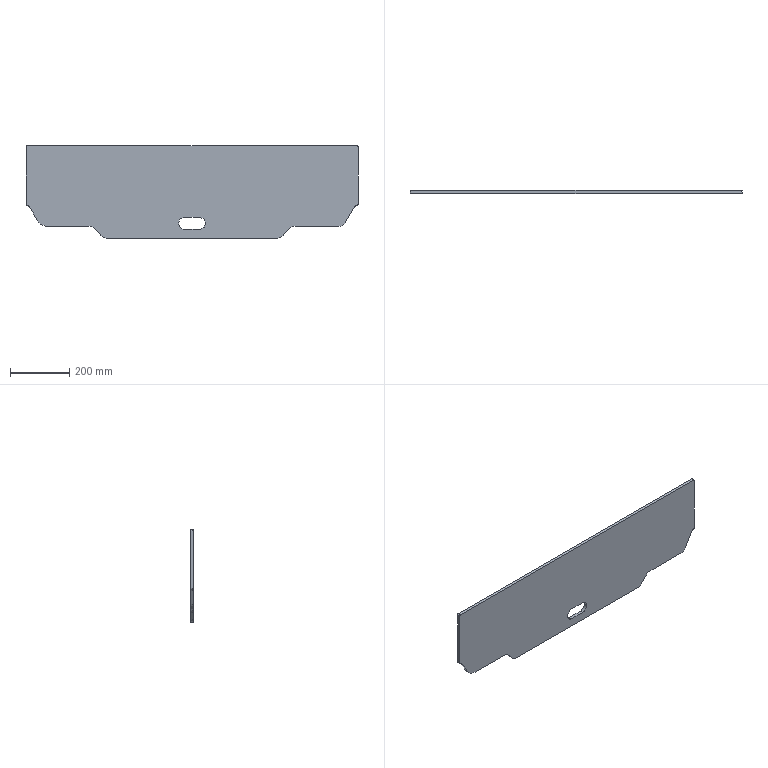Component | SolidWorks | FrontEndPlate,2-1 | 1 solid | 31 faces | box 1122 x 10 x 311.54 mm | volume 3226206 mm3 | plane 16 | cylinder 15 | commonest cylinder face diameters 50 x5 6 x4 40 x3 20 x2 80 x1 | material Q235
build123d program:
from build123d import *

# Parameters (mm, degrees)
BOSS_EXTRUDE1_DEPTH = 10


with BuildPart() as part:
    # Sketch1 → Boss-Extrude1 (new body)
    with BuildSketch(Plane.XY):
        with BuildLine():
            ThreePointArc((-290.657, -208.921), (-280.719, -210.981), (-272.419, -216.822))
            Line((-272.419, -216.822), (-249.734, -241.019))
            ThreePointArc((-249.734, -241.019), (-241.434, -246.861), (-231.495, -248.921))
            Line((-231.495, -248.921), (-59.652, -248.921))
            Line((-59.652, -248.921), (-13.084, -248.921))
            Line((-13.084, -248.921), (-2.185, -248.921))
            Line((-2.185, -248.921), (128.78, -248.921))
            Line((128.78, -248.921), (347.191, -248.921))
            ThreePointArc((347.191, -248.921), (357.129, -246.861), (365.43, -241.019))
            Line((365.43, -241.019), (388.114, -216.822))
            ThreePointArc((388.114, -216.822), (396.415, -210.981), (406.353, -208.921))
            Line((406.353, -208.921), (545.557, -208.921))
            ThreePointArc((545.557, -208.921), (565.355, -203.678), (579.962, -189.324))
            Line((579.962, -189.324), (607.86, -142.281))
            ThreePointArc((607.86, -142.281), (611.512, -138.692), (616.461, -137.382))
            Line((616.461, -137.382), (615.843, -137.382))
            ThreePointArc((615.843, -137.382), (617.964, -136.503), (618.843, -134.382))
            Line((618.843, -134.382), (618.843, 59.618))
            ThreePointArc((618.843, 59.618), (617.964, 61.74), (615.843, 62.618))
            Line((615.843, 62.618), (-240.657, 62.618))
            Line((-240.657, 62.618), (-500.157, 62.618))
            ThreePointArc((-500.157, 62.618), (-502.278, 61.74), (-503.157, 59.618))
            Line((-503.157, 59.618), (-503.157, -134.382))
            ThreePointArc((-503.157, -134.382), (-502.278, -136.503), (-500.157, -137.382))
            Line((-500.157, -137.382), (-500.765, -137.382))
            ThreePointArc((-500.765, -137.382), (-495.816, -138.692), (-492.164, -142.281))
            Line((-492.164, -142.281), (-460.397, -195.848))
            Line((-460.397, -195.848), (-459.43, -197.479))
            ThreePointArc((-459.43, -197.479), (-450.385, -205.875), (-438.426, -208.921))
            Line((-438.426, -208.921), (-290.657, -208.921))
        make_face()
        with BuildLine():
            ThreePointArc((32.848, -219.081), (12.85, -199.081), (32.848, -179.081))
            Line((32.848, -179.081), (82.848, -179.081))
            ThreePointArc((82.848, -179.081), (102.848, -199.081), (82.848, -219.081))
            Line((82.848, -219.081), (32.848, -219.081))
        make_face(mode=Mode.SUBTRACT)
    extrude(amount=BOSS_EXTRUDE1_DEPTH)


solid = part.part

# Placed as in the assembly
solid = solid.moved(Location((-759.311, 2402.474, 2748.087), (-90, 0, 180)))
STEP:
#1=COLOUR_RGB('',0.7922,0.8196,0.9333);
#2=FILL_AREA_STYLE_COLOUR('',#1);
#3=FILL_AREA_STYLE('',(#2));
#4=SURFACE_STYLE_FILL_AREA(#3);
#5=SURFACE_SIDE_STYLE('',(#4));
#6=SURFACE_STYLE_USAGE(.BOTH.,#5);
#7=PRESENTATION_STYLE_ASSIGNMENT((#6));
#8=CARTESIAN_POINT('',(-31.187,94.979,101.142));
#9=VERTEX_POINT('',#8);
#10=CARTESIAN_POINT('',(-30.4,94.979,100.355));
#11=VERTEX_POINT('',#10);
#12=CARTESIAN_POINT('',(-31.187,94.979,100.355));
#13=DIRECTION('',(-0.,1.,0.));
#14=DIRECTION('',(-1.,0.,0.));
#15=AXIS2_PLACEMENT_3D('',#12,#13,#14);
#16=CIRCLE('',#15,0.7874);
#17=EDGE_CURVE('',#9,#11,#16,.T.);
#18=ORIENTED_EDGE('',*,*,#17,.T.);
#19=CARTESIAN_POINT('',(-30.4,94.586,100.355));
#20=VERTEX_POINT('',#19);
#21=CARTESIAN_POINT('',(-30.4,94.979,100.355));
#22=DIRECTION('',(0.,-1.,-0.));
#23=VECTOR('',#22,39.37);
#24=LINE('',#21,#23);
#25=EDGE_CURVE('',#11,#20,#24,.T.);
#26=ORIENTED_EDGE('',*,*,#25,.T.);
#27=CARTESIAN_POINT('',(-31.187,94.586,101.142));
#28=VERTEX_POINT('',#27);
#29=CARTESIAN_POINT('',(-31.187,94.586,100.355));
#30=DIRECTION('',(-0.,1.,0.));
#31=DIRECTION('',(-1.,0.,0.));
#32=AXIS2_PLACEMENT_3D('',#29,#30,#31);
#33=CIRCLE('',#32,0.7874);
#34=EDGE_CURVE('',#28,#20,#33,.T.);
#35=ORIENTED_EDGE('',*,*,#34,.F.);
#36=CARTESIAN_POINT('',(-31.187,94.979,101.142));
#37=DIRECTION('',(0.,-1.,-0.));
#38=VECTOR('',#37,39.37);
#39=LINE('',#36,#38);
#40=EDGE_CURVE('',#9,#28,#39,.T.);
#41=ORIENTED_EDGE('',*,*,#40,.F.);
#42=EDGE_LOOP('',(#18,#26,#35,#41));
#43=FACE_OUTER_BOUND('',#42,.T.);
#44=CARTESIAN_POINT('',(-31.187,94.979,100.355));
#45=DIRECTION('',(0.,-1.,-0.));
#46=DIRECTION('',(1.,0.,-0.));
#47=AXIS2_PLACEMENT_3D('',#44,#45,#46);
#48=CYLINDRICAL_SURFACE('',#47,0.7874);
#49=ADVANCED_FACE('',(#43),#48,.F.);
#50=CARTESIAN_POINT('',(-54.258,94.586,110.54));
#51=VERTEX_POINT('',#50);
#52=CARTESIAN_POINT('',(-54.258,94.586,102.902));
#53=VERTEX_POINT('',#52);
#54=CARTESIAN_POINT('',(-54.258,94.586,108.192));
#55=DIRECTION('',(-0.,0.,-1.));
#56=VECTOR('',#55,39.37);
#57=LINE('',#54,#56);
#58=EDGE_CURVE('',#51,#53,#57,.T.);
#59=ORIENTED_EDGE('',*,*,#58,.F.);
#60=CARTESIAN_POINT('',(-54.258,94.979,110.54));
#61=VERTEX_POINT('',#60);
#62=CARTESIAN_POINT('',(-54.258,94.979,110.54));
#63=DIRECTION('',(0.,-1.,-0.));
#64=VECTOR('',#63,39.37);
#65=LINE('',#62,#64);
#66=EDGE_CURVE('',#61,#51,#65,.T.);
#67=ORIENTED_EDGE('',*,*,#66,.F.);
#68=CARTESIAN_POINT('',(-54.258,94.979,102.902));
#69=VERTEX_POINT('',#68);
#70=CARTESIAN_POINT('',(-54.258,94.979,108.192));
#71=DIRECTION('',(-0.,0.,-1.));
#72=VECTOR('',#71,39.37);
#73=LINE('',#70,#72);
#74=EDGE_CURVE('',#61,#69,#73,.T.);
#75=ORIENTED_EDGE('',*,*,#74,.T.);
#76=CARTESIAN_POINT('',(-54.258,94.979,102.902));
#77=DIRECTION('',(0.,-1.,-0.));
#78=VECTOR('',#77,39.37);
#79=LINE('',#76,#78);
#80=EDGE_CURVE('',#69,#53,#79,.T.);
#81=ORIENTED_EDGE('',*,*,#80,.T.);
#82=EDGE_LOOP('',(#59,#67,#75,#81));
#83=FACE_OUTER_BOUND('',#82,.T.);
#84=CARTESIAN_POINT('',(-54.258,94.979,108.192));
#85=DIRECTION('',(-1.,-0.,0.));
#86=DIRECTION('',(0.,-1.,-0.));
#87=AXIS2_PLACEMENT_3D('',#84,#85,#86);
#88=PLANE('',#87);
#89=ADVANCED_FACE('',(#83),#88,.T.);
#90=CARTESIAN_POINT('',(-54.14,94.586,110.658));
#91=VERTEX_POINT('',#90);
#92=CARTESIAN_POINT('',(-54.14,94.586,110.54));
#93=DIRECTION('',(-0.,1.,0.));
#94=DIRECTION('',(-1.,0.,0.));
#95=AXIS2_PLACEMENT_3D('',#92,#93,#94);
#96=CIRCLE('',#95,0.1181);
#97=EDGE_CURVE('',#51,#91,#96,.T.);
#98=ORIENTED_EDGE('',*,*,#97,.T.);
#99=CARTESIAN_POINT('',(-54.14,94.979,110.658));
#100=VERTEX_POINT('',#99);
#101=CARTESIAN_POINT('',(-54.14,94.979,110.658));
#102=DIRECTION('',(0.,-1.,-0.));
#103=VECTOR('',#102,39.37);
#104=LINE('',#101,#103);
#105=EDGE_CURVE('',#100,#91,#104,.T.);
#106=ORIENTED_EDGE('',*,*,#105,.F.);
#107=CARTESIAN_POINT('',(-54.14,94.979,110.54));
#108=DIRECTION('',(-0.,1.,0.));
#109=DIRECTION('',(-1.,0.,0.));
#110=AXIS2_PLACEMENT_3D('',#107,#108,#109);
#111=CIRCLE('',#110,0.1181);
#112=EDGE_CURVE('',#61,#100,#111,.T.);
#113=ORIENTED_EDGE('',*,*,#112,.F.);
#114=ORIENTED_EDGE('',*,*,#66,.T.);
#115=EDGE_LOOP('',(#98,#106,#113,#114));
#116=FACE_OUTER_BOUND('',#115,.T.);
#117=CARTESIAN_POINT('',(-54.14,94.979,110.54));
#118=DIRECTION('',(0.,-1.,-0.));
#119=DIRECTION('',(1.,0.,0.));
#120=AXIS2_PLACEMENT_3D('',#117,#118,#119);
#121=CYLINDRICAL_SURFACE('',#120,0.1181);
#122=ADVANCED_FACE('',(#116),#121,.T.);
#123=CARTESIAN_POINT('',(-10.203,94.586,110.658));
#124=VERTEX_POINT('',#123);
#125=CARTESIAN_POINT('',(-29.894,94.586,110.658));
#126=DIRECTION('',(1.,0.,-0.));
#127=VECTOR('',#126,39.37);
#128=LINE('',#125,#127);
#129=EDGE_CURVE('',#91,#124,#128,.T.);
#130=ORIENTED_EDGE('',*,*,#129,.T.);
#131=CARTESIAN_POINT('',(-10.203,94.979,110.658));
#132=VERTEX_POINT('',#131);
#133=CARTESIAN_POINT('',(-10.203,94.979,110.658));
#134=DIRECTION('',(0.,-1.,-0.));
#135=VECTOR('',#134,39.37);
#136=LINE('',#133,#135);
#137=EDGE_CURVE('',#132,#124,#136,.T.);
#138=ORIENTED_EDGE('',*,*,#137,.F.);
#139=CARTESIAN_POINT('',(-29.894,94.979,110.658));
#140=DIRECTION('',(1.,0.,-0.));
#141=VECTOR('',#140,39.37);
#142=LINE('',#139,#141);
#143=EDGE_CURVE('',#100,#132,#142,.T.);
#144=ORIENTED_EDGE('',*,*,#143,.F.);
#145=ORIENTED_EDGE('',*,*,#105,.T.);
#146=EDGE_LOOP('',(#130,#138,#144,#145));
#147=FACE_OUTER_BOUND('',#146,.T.);
#148=CARTESIAN_POINT('',(-29.894,94.979,110.658));
#149=DIRECTION('',(-0.,0.,-1.));
#150=DIRECTION('',(0.,-1.,-0.));
#151=AXIS2_PLACEMENT_3D('',#148,#149,#150);
#152=PLANE('',#151);
#153=ADVANCED_FACE('',(#147),#152,.F.);
#154=CARTESIAN_POINT('',(-10.085,94.586,110.54));
#155=VERTEX_POINT('',#154);
#156=CARTESIAN_POINT('',(-10.203,94.586,110.54));
#157=DIRECTION('',(-0.,1.,0.));
#158=DIRECTION('',(-1.,0.,0.));
#159=AXIS2_PLACEMENT_3D('',#156,#157,#158);
#160=CIRCLE('',#159,0.1181);
#161=EDGE_CURVE('',#124,#155,#160,.T.);
#162=ORIENTED_EDGE('',*,*,#161,.T.);
#163=CARTESIAN_POINT('',(-10.085,94.979,110.54));
#164=VERTEX_POINT('',#163);
#165=CARTESIAN_POINT('',(-10.085,94.979,110.54));
#166=DIRECTION('',(0.,-1.,-0.));
#167=VECTOR('',#166,39.37);
#168=LINE('',#165,#167);
#169=EDGE_CURVE('',#164,#155,#168,.T.);
#170=ORIENTED_EDGE('',*,*,#169,.F.);
#171=CARTESIAN_POINT('',(-10.203,94.979,110.54));
#172=DIRECTION('',(-0.,1.,0.));
#173=DIRECTION('',(-1.,0.,0.));
#174=AXIS2_PLACEMENT_3D('',#171,#172,#173);
#175=CIRCLE('',#174,0.1181);
#176=EDGE_CURVE('',#132,#164,#175,.T.);
#177=ORIENTED_EDGE('',*,*,#176,.F.);
#178=ORIENTED_EDGE('',*,*,#137,.T.);
#179=EDGE_LOOP('',(#162,#170,#177,#178));
#180=FACE_OUTER_BOUND('',#179,.T.);
#181=CARTESIAN_POINT('',(-10.203,94.979,110.54));
#182=DIRECTION('',(0.,-1.,-0.));
#183=DIRECTION('',(1.,0.,0.));
#184=AXIS2_PLACEMENT_3D('',#181,#182,#183);
#185=CYLINDRICAL_SURFACE('',#184,0.1181);
#186=ADVANCED_FACE('',(#180),#185,.T.);
#187=CARTESIAN_POINT('',(-10.085,94.586,102.902));
#188=VERTEX_POINT('',#187);
#189=CARTESIAN_POINT('',(-10.085,94.586,108.192));
#190=DIRECTION('',(0.,0.,-1.));
#191=VECTOR('',#190,39.37);
#192=LINE('',#189,#191);
#193=EDGE_CURVE('',#155,#188,#192,.T.);
#194=ORIENTED_EDGE('',*,*,#193,.T.);
#195=CARTESIAN_POINT('',(-10.085,94.979,102.902));
#196=VERTEX_POINT('',#195);
#197=CARTESIAN_POINT('',(-10.085,94.979,102.902));
#198=DIRECTION('',(0.,-1.,-0.));
#199=VECTOR('',#198,39.37);
#200=LINE('',#197,#199);
#201=EDGE_CURVE('',#196,#188,#200,.T.);
#202=ORIENTED_EDGE('',*,*,#201,.F.);
#203=CARTESIAN_POINT('',(-10.085,94.979,108.192));
#204=DIRECTION('',(0.,0.,-1.));
#205=VECTOR('',#204,39.37);
#206=LINE('',#203,#205);
#207=EDGE_CURVE('',#164,#196,#206,.T.);
#208=ORIENTED_EDGE('',*,*,#207,.F.);
#209=ORIENTED_EDGE('',*,*,#169,.T.);
#210=EDGE_LOOP('',(#194,#202,#208,#209));
#211=FACE_OUTER_BOUND('',#210,.T.);
#212=CARTESIAN_POINT('',(-10.085,94.979,108.192));
#213=DIRECTION('',(-1.,-0.,-0.));
#214=DIRECTION('',(-0.,-0.,1.));
#215=AXIS2_PLACEMENT_3D('',#212,#213,#214);
#216=PLANE('',#215);
#217=ADVANCED_FACE('',(#211),#216,.F.);
#218=CARTESIAN_POINT('',(-10.203,94.586,102.784));
#219=VERTEX_POINT('',#218);
#220=CARTESIAN_POINT('',(-10.203,94.586,102.902));
#221=DIRECTION('',(-0.,1.,0.));
#222=DIRECTION('',(-1.,0.,0.));
#223=AXIS2_PLACEMENT_3D('',#220,#221,#222);
#224=CIRCLE('',#223,0.1181);
#225=EDGE_CURVE('',#188,#219,#224,.T.);
#226=ORIENTED_EDGE('',*,*,#225,.T.);
#227=CARTESIAN_POINT('',(-10.203,94.979,102.784));
#228=VERTEX_POINT('',#227);
#229=CARTESIAN_POINT('',(-10.203,94.979,102.784));
#230=DIRECTION('',(0.,-1.,-0.));
#231=VECTOR('',#230,39.37);
#232=LINE('',#229,#231);
#233=EDGE_CURVE('',#228,#219,#232,.T.);
#234=ORIENTED_EDGE('',*,*,#233,.F.);
#235=CARTESIAN_POINT('',(-10.203,94.979,102.902));
#236=DIRECTION('',(-0.,1.,0.));
#237=DIRECTION('',(-1.,0.,0.));
#238=AXIS2_PLACEMENT_3D('',#235,#236,#237);
#239=CIRCLE('',#238,0.1181);
#240=EDGE_CURVE('',#196,#228,#239,.T.);
#241=ORIENTED_EDGE('',*,*,#240,.F.);
#242=ORIENTED_EDGE('',*,*,#201,.T.);
#243=EDGE_LOOP('',(#226,#234,#241,#242));
#244=FACE_OUTER_BOUND('',#243,.T.);
#245=CARTESIAN_POINT('',(-10.203,94.979,102.902));
#246=DIRECTION('',(0.,-1.,-0.));
#247=DIRECTION('',(1.,0.,0.));
#248=AXIS2_PLACEMENT_3D('',#245,#246,#247);
#249=CYLINDRICAL_SURFACE('',#248,0.1181);
#250=ADVANCED_FACE('',(#244),#249,.T.);
#251=CARTESIAN_POINT('',(-10.179,94.586,102.784));
#252=VERTEX_POINT('',#251);
#253=CARTESIAN_POINT('',(-29.894,94.586,102.784));
#254=DIRECTION('',(1.,0.,-0.));
#255=VECTOR('',#254,39.37);
#256=LINE('',#253,#255);
#257=EDGE_CURVE('',#219,#252,#256,.T.);
#258=ORIENTED_EDGE('',*,*,#257,.T.);
#259=CARTESIAN_POINT('',(-10.179,94.979,102.784));
#260=VERTEX_POINT('',#259);
#261=CARTESIAN_POINT('',(-10.179,94.979,102.784));
#262=DIRECTION('',(0.,-1.,-0.));
#263=VECTOR('',#262,39.37);
#264=LINE('',#261,#263);
#265=EDGE_CURVE('',#260,#252,#264,.T.);
#266=ORIENTED_EDGE('',*,*,#265,.F.);
#267=CARTESIAN_POINT('',(-29.894,94.979,102.784));
#268=DIRECTION('',(1.,0.,-0.));
#269=VECTOR('',#268,39.37);
#270=LINE('',#267,#269);
#271=EDGE_CURVE('',#228,#260,#270,.T.);
#272=ORIENTED_EDGE('',*,*,#271,.F.);
#273=ORIENTED_EDGE('',*,*,#233,.T.);
#274=EDGE_LOOP('',(#258,#266,#272,#273));
#275=FACE_OUTER_BOUND('',#274,.T.);
#276=CARTESIAN_POINT('',(-29.894,94.979,102.784));
#277=DIRECTION('',(-0.,0.,-1.));
#278=DIRECTION('',(0.,-1.,-0.));
#279=AXIS2_PLACEMENT_3D('',#276,#277,#278);
#280=PLANE('',#279);
#281=ADVANCED_FACE('',(#275),#280,.F.);
#282=CARTESIAN_POINT('',(-10.518,94.586,102.591));
#283=VERTEX_POINT('',#282);
#284=CARTESIAN_POINT('',(-10.179,94.586,102.39));
#285=DIRECTION('',(-0.,1.,0.));
#286=DIRECTION('',(-1.,0.,0.));
#287=AXIS2_PLACEMENT_3D('',#284,#285,#286);
#288=CIRCLE('',#287,0.3937);
#289=EDGE_CURVE('',#283,#252,#288,.T.);
#290=ORIENTED_EDGE('',*,*,#289,.F.);
#291=CARTESIAN_POINT('',(-10.518,94.979,102.591));
#292=VERTEX_POINT('',#291);
#293=CARTESIAN_POINT('',(-10.518,94.979,102.591));
#294=DIRECTION('',(0.,-1.,-0.));
#295=VECTOR('',#294,39.37);
#296=LINE('',#293,#295);
#297=EDGE_CURVE('',#292,#283,#296,.T.);
#298=ORIENTED_EDGE('',*,*,#297,.F.);
#299=CARTESIAN_POINT('',(-10.179,94.979,102.39));
#300=DIRECTION('',(-0.,1.,0.));
#301=DIRECTION('',(-1.,0.,0.));
#302=AXIS2_PLACEMENT_3D('',#299,#300,#301);
#303=CIRCLE('',#302,0.3937);
#304=EDGE_CURVE('',#292,#260,#303,.T.);
#305=ORIENTED_EDGE('',*,*,#304,.T.);
#306=ORIENTED_EDGE('',*,*,#265,.T.);
#307=EDGE_LOOP('',(#290,#298,#305,#306));
#308=FACE_OUTER_BOUND('',#307,.T.);
#309=CARTESIAN_POINT('',(-10.179,94.979,102.39));
#310=DIRECTION('',(0.,-1.,-0.));
#311=DIRECTION('',(1.,0.,0.));
#312=AXIS2_PLACEMENT_3D('',#309,#310,#311);
#313=CYLINDRICAL_SURFACE('',#312,0.3937);
#314=ADVANCED_FACE('',(#308),#313,.F.);
#315=CARTESIAN_POINT('',(-11.806,94.586,100.418));
#316=VERTEX_POINT('',#315);
#317=CARTESIAN_POINT('',(-13.101,94.586,98.234));
#318=DIRECTION('',(-0.5101,-0.,-0.8601));
#319=VECTOR('',#318,39.37);
#320=LINE('',#317,#319);
#321=EDGE_CURVE('',#283,#316,#320,.T.);
#322=ORIENTED_EDGE('',*,*,#321,.T.);
#323=CARTESIAN_POINT('',(-11.806,94.979,100.418));
#324=VERTEX_POINT('',#323);
#325=CARTESIAN_POINT('',(-11.806,94.979,100.418));
#326=DIRECTION('',(0.,-1.,-0.));
#327=VECTOR('',#326,39.37);
#328=LINE('',#325,#327);
#329=EDGE_CURVE('',#324,#316,#328,.T.);
#330=ORIENTED_EDGE('',*,*,#329,.F.);
#331=CARTESIAN_POINT('',(-13.101,94.979,98.234));
#332=DIRECTION('',(-0.5101,-0.,-0.8601));
#333=VECTOR('',#332,39.37);
#334=LINE('',#331,#333);
#335=EDGE_CURVE('',#292,#324,#334,.T.);
#336=ORIENTED_EDGE('',*,*,#335,.F.);
#337=ORIENTED_EDGE('',*,*,#297,.T.);
#338=EDGE_LOOP('',(#322,#330,#336,#337));
#339=FACE_OUTER_BOUND('',#338,.T.);
#340=CARTESIAN_POINT('',(-13.101,94.979,98.234));
#341=DIRECTION('',(-0.8601,-0.,0.5101));
#342=DIRECTION('',(0.5101,0.,0.8601));
#343=AXIS2_PLACEMENT_3D('',#340,#341,#342);
#344=PLANE('',#343);
#345=ADVANCED_FACE('',(#339),#344,.F.);
#346=CARTESIAN_POINT('',(-12.633,94.586,99.967));
#347=VERTEX_POINT('',#346);
#348=CARTESIAN_POINT('',(-12.633,94.586,100.951));
#349=DIRECTION('',(-0.,1.,0.));
#350=DIRECTION('',(-1.,-0.,0.));
#351=AXIS2_PLACEMENT_3D('',#348,#349,#350);
#352=CIRCLE('',#351,0.9843);
#353=EDGE_CURVE('',#316,#347,#352,.T.);
#354=ORIENTED_EDGE('',*,*,#353,.T.);
#355=CARTESIAN_POINT('',(-12.633,94.979,99.967));
#356=VERTEX_POINT('',#355);
#357=CARTESIAN_POINT('',(-12.633,94.979,99.967));
#358=DIRECTION('',(0.,-1.,-0.));
#359=VECTOR('',#358,39.37);
#360=LINE('',#357,#359);
#361=EDGE_CURVE('',#356,#347,#360,.T.);
#362=ORIENTED_EDGE('',*,*,#361,.F.);
#363=CARTESIAN_POINT('',(-12.633,94.979,100.951));
#364=DIRECTION('',(-0.,1.,0.));
#365=DIRECTION('',(-1.,-0.,0.));
#366=AXIS2_PLACEMENT_3D('',#363,#364,#365);
#367=CIRCLE('',#366,0.9843);
#368=EDGE_CURVE('',#324,#356,#367,.T.);
#369=ORIENTED_EDGE('',*,*,#368,.F.);
#370=ORIENTED_EDGE('',*,*,#329,.T.);
#371=EDGE_LOOP('',(#354,#362,#369,#370));
#372=FACE_OUTER_BOUND('',#371,.T.);
#373=CARTESIAN_POINT('',(-12.633,94.979,100.951));
#374=DIRECTION('',(0.,-1.,-0.));
#375=DIRECTION('',(1.,0.,-0.));
#376=AXIS2_PLACEMENT_3D('',#373,#374,#375);
#377=CYLINDRICAL_SURFACE('',#376,0.9843);
#378=ADVANCED_FACE('',(#372),#377,.T.);
#379=CARTESIAN_POINT('',(-18.451,94.586,99.967));
#380=VERTEX_POINT('',#379);
#381=CARTESIAN_POINT('',(-29.894,94.586,99.967));
#382=DIRECTION('',(-1.,-0.,0.));
#383=VECTOR('',#382,39.37);
#384=LINE('',#381,#383);
#385=EDGE_CURVE('',#347,#380,#384,.T.);
#386=ORIENTED_EDGE('',*,*,#385,.T.);
#387=CARTESIAN_POINT('',(-18.451,94.979,99.967));
#388=VERTEX_POINT('',#387);
#389=CARTESIAN_POINT('',(-18.451,94.979,99.967));
#390=DIRECTION('',(0.,-1.,-0.));
#391=VECTOR('',#390,39.37);
#392=LINE('',#389,#391);
#393=EDGE_CURVE('',#388,#380,#392,.T.);
#394=ORIENTED_EDGE('',*,*,#393,.F.);
#395=CARTESIAN_POINT('',(-29.894,94.979,99.967));
#396=DIRECTION('',(-1.,-0.,0.));
#397=VECTOR('',#396,39.37);
#398=LINE('',#395,#397);
#399=EDGE_CURVE('',#356,#388,#398,.T.);
#400=ORIENTED_EDGE('',*,*,#399,.F.);
#401=ORIENTED_EDGE('',*,*,#361,.T.);
#402=EDGE_LOOP('',(#386,#394,#400,#401));
#403=FACE_OUTER_BOUND('',#402,.T.);
#404=CARTESIAN_POINT('',(-29.894,94.979,99.967));
#405=DIRECTION('',(0.,-0.,1.));
#406=DIRECTION('',(1.,0.,-0.));
#407=AXIS2_PLACEMENT_3D('',#404,#405,#406);
#408=PLANE('',#407);
#409=ADVANCED_FACE('',(#403),#408,.F.);
#410=CARTESIAN_POINT('',(-19.169,94.586,99.656));
#411=VERTEX_POINT('',#410);
#412=CARTESIAN_POINT('',(-18.451,94.586,98.983));
#413=DIRECTION('',(-0.,1.,0.));
#414=DIRECTION('',(-1.,-0.,0.));
#415=AXIS2_PLACEMENT_3D('',#412,#413,#414);
#416=CIRCLE('',#415,0.9843);
#417=EDGE_CURVE('',#411,#380,#416,.T.);
#418=ORIENTED_EDGE('',*,*,#417,.F.);
#419=CARTESIAN_POINT('',(-19.169,94.979,99.656));
#420=VERTEX_POINT('',#419);
#421=CARTESIAN_POINT('',(-19.169,94.979,99.656));
#422=DIRECTION('',(0.,-1.,-0.));
#423=VECTOR('',#422,39.37);
#424=LINE('',#421,#423);
#425=EDGE_CURVE('',#420,#411,#424,.T.);
#426=ORIENTED_EDGE('',*,*,#425,.F.);
#427=CARTESIAN_POINT('',(-18.451,94.979,98.983));
#428=DIRECTION('',(-0.,1.,0.));
#429=DIRECTION('',(-1.,-0.,0.));
#430=AXIS2_PLACEMENT_3D('',#427,#428,#429);
#431=CIRCLE('',#430,0.9843);
#432=EDGE_CURVE('',#420,#388,#431,.T.);
#433=ORIENTED_EDGE('',*,*,#432,.T.);
#434=ORIENTED_EDGE('',*,*,#393,.T.);
#435=EDGE_LOOP('',(#418,#426,#433,#434));
#436=FACE_OUTER_BOUND('',#435,.T.);
#437=CARTESIAN_POINT('',(-18.451,94.979,98.983));
#438=DIRECTION('',(0.,-1.,-0.));
#439=DIRECTION('',(1.,0.,-0.));
#440=AXIS2_PLACEMENT_3D('',#437,#438,#439);
#441=CYLINDRICAL_SURFACE('',#440,0.9843);
#442=ADVANCED_FACE('',(#436),#441,.F.);
#443=CARTESIAN_POINT('',(-20.062,94.586,98.703));
#444=VERTEX_POINT('',#443);
#445=CARTESIAN_POINT('',(-19.927,94.586,98.848));
#446=DIRECTION('',(-0.6839,-0.,-0.7295));
#447=VECTOR('',#446,39.37);
#448=LINE('',#445,#447);
#449=EDGE_CURVE('',#411,#444,#448,.T.);
#450=ORIENTED_EDGE('',*,*,#449,.T.);
#451=CARTESIAN_POINT('',(-20.062,94.979,98.703));
#452=VERTEX_POINT('',#451);
#453=CARTESIAN_POINT('',(-20.062,94.979,98.703));
#454=DIRECTION('',(0.,-1.,-0.));
#455=VECTOR('',#454,39.37);
#456=LINE('',#453,#455);
#457=EDGE_CURVE('',#452,#444,#456,.T.);
#458=ORIENTED_EDGE('',*,*,#457,.F.);
#459=CARTESIAN_POINT('',(-19.927,94.979,98.848));
#460=DIRECTION('',(-0.6839,-0.,-0.7295));
#461=VECTOR('',#460,39.37);
#462=LINE('',#459,#461);
#463=EDGE_CURVE('',#420,#452,#462,.T.);
#464=ORIENTED_EDGE('',*,*,#463,.F.);
#465=ORIENTED_EDGE('',*,*,#425,.T.);
#466=EDGE_LOOP('',(#450,#458,#464,#465));
#467=FACE_OUTER_BOUND('',#466,.T.);
#468=CARTESIAN_POINT('',(-19.927,94.979,98.848));
#469=DIRECTION('',(-0.7295,-0.,0.6839));
#470=DIRECTION('',(0.6839,0.,0.7295));
#471=AXIS2_PLACEMENT_3D('',#468,#469,#470);
#472=PLANE('',#471);
#473=ADVANCED_FACE('',(#467),#472,.F.);
#474=CARTESIAN_POINT('',(-20.78,94.586,98.392));
#475=VERTEX_POINT('',#474);
#476=CARTESIAN_POINT('',(-20.78,94.586,99.377));
#477=DIRECTION('',(-0.,1.,0.));
#478=DIRECTION('',(-1.,-0.,0.));
#479=AXIS2_PLACEMENT_3D('',#476,#477,#478);
#480=CIRCLE('',#479,0.9843);
#481=EDGE_CURVE('',#444,#475,#480,.T.);
#482=ORIENTED_EDGE('',*,*,#481,.T.);
#483=CARTESIAN_POINT('',(-20.78,94.979,98.392));
#484=VERTEX_POINT('',#483);
#485=CARTESIAN_POINT('',(-20.78,94.979,98.392));
#486=DIRECTION('',(0.,-1.,-0.));
#487=VECTOR('',#486,39.37);
#488=LINE('',#485,#487);
#489=EDGE_CURVE('',#484,#475,#488,.T.);
#490=ORIENTED_EDGE('',*,*,#489,.F.);
#491=CARTESIAN_POINT('',(-20.78,94.979,99.377));
#492=DIRECTION('',(-0.,1.,0.));
#493=DIRECTION('',(-1.,-0.,0.));
#494=AXIS2_PLACEMENT_3D('',#491,#492,#493);
#495=CIRCLE('',#494,0.9843);
#496=EDGE_CURVE('',#452,#484,#495,.T.);
#497=ORIENTED_EDGE('',*,*,#496,.F.);
#498=ORIENTED_EDGE('',*,*,#457,.T.);
#499=EDGE_LOOP('',(#482,#490,#497,#498));
#500=FACE_OUTER_BOUND('',#499,.T.);
#501=CARTESIAN_POINT('',(-20.78,94.979,99.377));
#502=DIRECTION('',(0.,-1.,-0.));
#503=DIRECTION('',(1.,0.,-0.));
#504=AXIS2_PLACEMENT_3D('',#501,#502,#503);
#505=CYLINDRICAL_SURFACE('',#504,0.9843);
#506=ADVANCED_FACE('',(#500),#505,.T.);
#507=CARTESIAN_POINT('',(-43.563,94.586,98.392));
#508=VERTEX_POINT('',#507);
#509=CARTESIAN_POINT('',(-29.894,94.586,98.392));
#510=DIRECTION('',(-1.,-0.,0.));
#511=VECTOR('',#510,39.37);
#512=LINE('',#509,#511);
#513=EDGE_CURVE('',#475,#508,#512,.T.);
#514=ORIENTED_EDGE('',*,*,#513,.T.);
#515=CARTESIAN_POINT('',(-43.563,94.979,98.392));
#516=VERTEX_POINT('',#515);
#517=CARTESIAN_POINT('',(-43.563,94.979,98.392));
#518=DIRECTION('',(0.,-1.,-0.));
#519=VECTOR('',#518,39.37);
#520=LINE('',#517,#519);
#521=EDGE_CURVE('',#516,#508,#520,.T.);
#522=ORIENTED_EDGE('',*,*,#521,.F.);
#523=CARTESIAN_POINT('',(-29.894,94.979,98.392));
#524=DIRECTION('',(-1.,-0.,0.));
#525=VECTOR('',#524,39.37);
#526=LINE('',#523,#525);
#527=EDGE_CURVE('',#484,#516,#526,.T.);
#528=ORIENTED_EDGE('',*,*,#527,.F.);
#529=ORIENTED_EDGE('',*,*,#489,.T.);
#530=EDGE_LOOP('',(#514,#522,#528,#529));
#531=FACE_OUTER_BOUND('',#530,.T.);
#532=CARTESIAN_POINT('',(-29.894,94.979,98.392));
#533=DIRECTION('',(0.,-0.,1.));
#534=DIRECTION('',(1.,0.,-0.));
#535=AXIS2_PLACEMENT_3D('',#532,#533,#534);
#536=PLANE('',#535);
#537=ADVANCED_FACE('',(#531),#536,.F.);
#538=CARTESIAN_POINT('',(-44.281,94.586,98.703));
#539=VERTEX_POINT('',#538);
#540=CARTESIAN_POINT('',(-43.563,94.586,99.377));
#541=DIRECTION('',(-0.,1.,0.));
#542=DIRECTION('',(-1.,-0.,0.));
#543=AXIS2_PLACEMENT_3D('',#540,#541,#542);
#544=CIRCLE('',#543,0.9843);
#545=EDGE_CURVE('',#508,#539,#544,.T.);
#546=ORIENTED_EDGE('',*,*,#545,.T.);
#547=CARTESIAN_POINT('',(-44.281,94.979,98.703));
#548=VERTEX_POINT('',#547);
#549=CARTESIAN_POINT('',(-44.281,94.979,98.703));
#550=DIRECTION('',(0.,-1.,-0.));
#551=VECTOR('',#550,39.37);
#552=LINE('',#549,#551);
#553=EDGE_CURVE('',#548,#539,#552,.T.);
#554=ORIENTED_EDGE('',*,*,#553,.F.);
#555=CARTESIAN_POINT('',(-43.563,94.979,99.377));
#556=DIRECTION('',(-0.,1.,0.));
#557=DIRECTION('',(-1.,-0.,0.));
#558=AXIS2_PLACEMENT_3D('',#555,#556,#557);
#559=CIRCLE('',#558,0.9843);
#560=EDGE_CURVE('',#516,#548,#559,.T.);
#561=ORIENTED_EDGE('',*,*,#560,.F.);
#562=ORIENTED_EDGE('',*,*,#521,.T.);
#563=EDGE_LOOP('',(#546,#554,#561,#562));
#564=FACE_OUTER_BOUND('',#563,.T.);
#565=CARTESIAN_POINT('',(-43.563,94.979,99.377));
#566=DIRECTION('',(0.,-1.,-0.));
#567=DIRECTION('',(1.,0.,-0.));
#568=AXIS2_PLACEMENT_3D('',#565,#566,#567);
#569=CYLINDRICAL_SURFACE('',#568,0.9843);
#570=ADVANCED_FACE('',(#564),#569,.T.);
#571=CARTESIAN_POINT('',(-45.174,94.586,99.656));
#572=VERTEX_POINT('',#571);
#573=CARTESIAN_POINT('',(-42.286,94.586,96.575));
#574=DIRECTION('',(0.6839,0.,-0.7295));
#575=VECTOR('',#574,39.37);
#576=LINE('',#573,#575);
#577=EDGE_CURVE('',#572,#539,#576,.T.);
#578=ORIENTED_EDGE('',*,*,#577,.F.);
#579=CARTESIAN_POINT('',(-45.174,94.979,99.656));
#580=VERTEX_POINT('',#579);
#581=CARTESIAN_POINT('',(-45.174,94.979,99.656));
#582=DIRECTION('',(0.,-1.,-0.));
#583=VECTOR('',#582,39.37);
#584=LINE('',#581,#583);
#585=EDGE_CURVE('',#580,#572,#584,.T.);
#586=ORIENTED_EDGE('',*,*,#585,.F.);
#587=CARTESIAN_POINT('',(-42.286,94.979,96.575));
#588=DIRECTION('',(0.6839,0.,-0.7295));
#589=VECTOR('',#588,39.37);
#590=LINE('',#587,#589);
#591=EDGE_CURVE('',#580,#548,#590,.T.);
#592=ORIENTED_EDGE('',*,*,#591,.T.);
#593=ORIENTED_EDGE('',*,*,#553,.T.);
#594=EDGE_LOOP('',(#578,#586,#592,#593));
#595=FACE_OUTER_BOUND('',#594,.T.);
#596=CARTESIAN_POINT('',(-42.286,94.979,96.575));
#597=DIRECTION('',(-0.7295,-0.,-0.6839));
#598=DIRECTION('',(-0.6839,-0.,0.7295));
#599=AXIS2_PLACEMENT_3D('',#596,#597,#598);
#600=PLANE('',#599);
#601=ADVANCED_FACE('',(#595),#600,.T.);
#602=CARTESIAN_POINT('',(-45.892,94.586,99.967));
#603=VERTEX_POINT('',#602);
#604=CARTESIAN_POINT('',(-45.892,94.586,98.983));
#605=DIRECTION('',(-0.,1.,0.));
#606=DIRECTION('',(-1.,-0.,0.));
#607=AXIS2_PLACEMENT_3D('',#604,#605,#606);
#608=CIRCLE('',#607,0.9843);
#609=EDGE_CURVE('',#603,#572,#608,.T.);
#610=ORIENTED_EDGE('',*,*,#609,.F.);
#611=CARTESIAN_POINT('',(-45.892,94.979,99.967));
#612=VERTEX_POINT('',#611);
#613=CARTESIAN_POINT('',(-45.892,94.979,99.967));
#614=DIRECTION('',(0.,-1.,-0.));
#615=VECTOR('',#614,39.37);
#616=LINE('',#613,#615);
#617=EDGE_CURVE('',#612,#603,#616,.T.);
#618=ORIENTED_EDGE('',*,*,#617,.F.);
#619=CARTESIAN_POINT('',(-45.892,94.979,98.983));
#620=DIRECTION('',(-0.,1.,0.));
#621=DIRECTION('',(-1.,-0.,0.));
#622=AXIS2_PLACEMENT_3D('',#619,#620,#621);
#623=CIRCLE('',#622,0.9843);
#624=EDGE_CURVE('',#612,#580,#623,.T.);
#625=ORIENTED_EDGE('',*,*,#624,.T.);
#626=ORIENTED_EDGE('',*,*,#585,.T.);
#627=EDGE_LOOP('',(#610,#618,#625,#626));
#628=FACE_OUTER_BOUND('',#627,.T.);
#629=CARTESIAN_POINT('',(-45.892,94.979,98.983));
#630=DIRECTION('',(0.,-1.,-0.));
#631=DIRECTION('',(1.,0.,-0.));
#632=AXIS2_PLACEMENT_3D('',#629,#630,#631);
#633=CYLINDRICAL_SURFACE('',#632,0.9843);
#634=ADVANCED_FACE('',(#628),#633,.F.);
#635=CARTESIAN_POINT('',(-51.373,94.586,99.967));
#636=VERTEX_POINT('',#635);
#637=CARTESIAN_POINT('',(-29.894,94.586,99.967));
#638=DIRECTION('',(1.,0.,-0.));
#639=VECTOR('',#638,39.37);
#640=LINE('',#637,#639);
#641=EDGE_CURVE('',#636,#603,#640,.T.);
#642=ORIENTED_EDGE('',*,*,#641,.F.);
#643=CARTESIAN_POINT('',(-51.373,94.979,99.967));
#644=VERTEX_POINT('',#643);
#645=CARTESIAN_POINT('',(-51.373,94.979,99.967));
#646=DIRECTION('',(0.,-1.,-0.));
#647=VECTOR('',#646,39.37);
#648=LINE('',#645,#647);
#649=EDGE_CURVE('',#644,#636,#648,.T.);
#650=ORIENTED_EDGE('',*,*,#649,.F.);
#651=CARTESIAN_POINT('',(-29.894,94.979,99.967));
#652=DIRECTION('',(1.,0.,-0.));
#653=VECTOR('',#652,39.37);
#654=LINE('',#651,#653);
#655=EDGE_CURVE('',#644,#612,#654,.T.);
#656=ORIENTED_EDGE('',*,*,#655,.T.);
#657=ORIENTED_EDGE('',*,*,#617,.T.);
#658=EDGE_LOOP('',(#642,#650,#656,#657));
#659=FACE_OUTER_BOUND('',#658,.T.);
#660=CARTESIAN_POINT('',(-29.894,94.979,99.967));
#661=DIRECTION('',(-0.,0.,-1.));
#662=DIRECTION('',(0.,-1.,-0.));
#663=AXIS2_PLACEMENT_3D('',#660,#661,#662);
#664=PLANE('',#663);
#665=ADVANCED_FACE('',(#659),#664,.T.);
#666=CARTESIAN_POINT('',(-52.727,94.586,100.739));
#667=VERTEX_POINT('',#666);
#668=CARTESIAN_POINT('',(-51.373,94.586,101.542));
#669=DIRECTION('',(-0.,1.,0.));
#670=DIRECTION('',(-1.,-0.,0.));
#671=AXIS2_PLACEMENT_3D('',#668,#669,#670);
#672=CIRCLE('',#671,1.575);
#673=EDGE_CURVE('',#636,#667,#672,.T.);
#674=ORIENTED_EDGE('',*,*,#673,.T.);
#675=CARTESIAN_POINT('',(-52.727,94.979,100.739));
#676=VERTEX_POINT('',#675);
#677=CARTESIAN_POINT('',(-52.727,94.979,100.739));
#678=DIRECTION('',(0.,-1.,-0.));
#679=VECTOR('',#678,39.37);
#680=LINE('',#677,#679);
#681=EDGE_CURVE('',#676,#667,#680,.T.);
#682=ORIENTED_EDGE('',*,*,#681,.F.);
#683=CARTESIAN_POINT('',(-51.373,94.979,101.542));
#684=DIRECTION('',(-0.,1.,0.));
#685=DIRECTION('',(-1.,-0.,0.));
#686=AXIS2_PLACEMENT_3D('',#683,#684,#685);
#687=CIRCLE('',#686,1.575);
#688=EDGE_CURVE('',#644,#676,#687,.T.);
#689=ORIENTED_EDGE('',*,*,#688,.F.);
#690=ORIENTED_EDGE('',*,*,#649,.T.);
#691=EDGE_LOOP('',(#674,#682,#689,#690));
#692=FACE_OUTER_BOUND('',#691,.T.);
#693=CARTESIAN_POINT('',(-51.373,94.979,101.542));
#694=DIRECTION('',(0.,-1.,-0.));
#695=DIRECTION('',(1.,0.,-0.));
#696=AXIS2_PLACEMENT_3D('',#693,#694,#695);
#697=CYLINDRICAL_SURFACE('',#696,1.575);
#698=ADVANCED_FACE('',(#692),#697,.T.);
#699=CARTESIAN_POINT('',(-53.826,94.586,102.591));
#700=VERTEX_POINT('',#699);
#701=CARTESIAN_POINT('',(-50.057,94.586,96.236));
#702=DIRECTION('',(0.5101,0.,-0.8601));
#703=VECTOR('',#702,39.37);
#704=LINE('',#701,#703);
#705=EDGE_CURVE('',#700,#667,#704,.T.);
#706=ORIENTED_EDGE('',*,*,#705,.F.);
#707=CARTESIAN_POINT('',(-53.826,94.979,102.591));
#708=VERTEX_POINT('',#707);
#709=CARTESIAN_POINT('',(-53.826,94.979,102.591));
#710=DIRECTION('',(0.,-1.,-0.));
#711=VECTOR('',#710,39.37);
#712=LINE('',#709,#711);
#713=EDGE_CURVE('',#708,#700,#712,.T.);
#714=ORIENTED_EDGE('',*,*,#713,.F.);
#715=CARTESIAN_POINT('',(-50.057,94.979,96.236));
#716=DIRECTION('',(0.5101,0.,-0.8601));
#717=VECTOR('',#716,39.37);
#718=LINE('',#715,#717);
#719=EDGE_CURVE('',#708,#676,#718,.T.);
#720=ORIENTED_EDGE('',*,*,#719,.T.);
#721=ORIENTED_EDGE('',*,*,#681,.T.);
#722=EDGE_LOOP('',(#706,#714,#720,#721));
#723=FACE_OUTER_BOUND('',#722,.T.);
#724=CARTESIAN_POINT('',(-50.057,94.979,96.236));
#725=DIRECTION('',(-0.8601,-0.,-0.5101));
#726=DIRECTION('',(-0.5101,-0.,0.8601));
#727=AXIS2_PLACEMENT_3D('',#724,#725,#726);
#728=PLANE('',#727);
#729=ADVANCED_FACE('',(#723),#728,.T.);
#730=CARTESIAN_POINT('',(-54.164,94.586,102.784));
#731=VERTEX_POINT('',#730);
#732=CARTESIAN_POINT('',(-54.164,94.586,102.39));
#733=DIRECTION('',(-0.,1.,0.));
#734=DIRECTION('',(-1.,0.,0.));
#735=AXIS2_PLACEMENT_3D('',#732,#733,#734);
#736=CIRCLE('',#735,0.3937);
#737=EDGE_CURVE('',#731,#700,#736,.T.);
#738=ORIENTED_EDGE('',*,*,#737,.F.);
#739=CARTESIAN_POINT('',(-54.164,94.979,102.784));
#740=VERTEX_POINT('',#739);
#741=CARTESIAN_POINT('',(-54.164,94.979,102.784));
#742=DIRECTION('',(0.,-1.,-0.));
#743=VECTOR('',#742,39.37);
#744=LINE('',#741,#743);
#745=EDGE_CURVE('',#740,#731,#744,.T.);
#746=ORIENTED_EDGE('',*,*,#745,.F.);
#747=CARTESIAN_POINT('',(-54.164,94.979,102.39));
#748=DIRECTION('',(-0.,1.,0.));
#749=DIRECTION('',(-1.,0.,0.));
#750=AXIS2_PLACEMENT_3D('',#747,#748,#749);
#751=CIRCLE('',#750,0.3937);
#752=EDGE_CURVE('',#740,#708,#751,.T.);
#753=ORIENTED_EDGE('',*,*,#752,.T.);
#754=ORIENTED_EDGE('',*,*,#713,.T.);
#755=EDGE_LOOP('',(#738,#746,#753,#754));
#756=FACE_OUTER_BOUND('',#755,.T.);
#757=CARTESIAN_POINT('',(-54.164,94.979,102.39));
#758=DIRECTION('',(0.,-1.,-0.));
#759=DIRECTION('',(1.,0.,0.));
#760=AXIS2_PLACEMENT_3D('',#757,#758,#759);
#761=CYLINDRICAL_SURFACE('',#760,0.3937);
#762=ADVANCED_FACE('',(#756),#761,.F.);
#763=CARTESIAN_POINT('',(-54.14,94.586,102.784));
#764=VERTEX_POINT('',#763);
#765=CARTESIAN_POINT('',(-29.894,94.586,102.784));
#766=DIRECTION('',(-1.,-0.,0.));
#767=VECTOR('',#766,39.37);
#768=LINE('',#765,#767);
#769=EDGE_CURVE('',#764,#731,#768,.T.);
#770=ORIENTED_EDGE('',*,*,#769,.F.);
#771=CARTESIAN_POINT('',(-54.14,94.979,102.784));
#772=VERTEX_POINT('',#771);
#773=CARTESIAN_POINT('',(-54.14,94.979,102.784));
#774=DIRECTION('',(0.,-1.,-0.));
#775=VECTOR('',#774,39.37);
#776=LINE('',#773,#775);
#777=EDGE_CURVE('',#772,#764,#776,.T.);
#778=ORIENTED_EDGE('',*,*,#777,.F.);
#779=CARTESIAN_POINT('',(-29.894,94.979,102.784));
#780=DIRECTION('',(-1.,-0.,0.));
#781=VECTOR('',#780,39.37);
#782=LINE('',#779,#781);
#783=EDGE_CURVE('',#772,#740,#782,.T.);
#784=ORIENTED_EDGE('',*,*,#783,.T.);
#785=ORIENTED_EDGE('',*,*,#745,.T.);
#786=EDGE_LOOP('',(#770,#778,#784,#785));
#787=FACE_OUTER_BOUND('',#786,.T.);
#788=CARTESIAN_POINT('',(-29.894,94.979,102.784));
#789=DIRECTION('',(0.,-0.,1.));
#790=DIRECTION('',(-0.,1.,0.));
#791=AXIS2_PLACEMENT_3D('',#788,#789,#790);
#792=PLANE('',#791);
#793=ADVANCED_FACE('',(#787),#792,.T.);
#794=CARTESIAN_POINT('',(-33.156,94.586,99.567));
#795=VERTEX_POINT('',#794);
#796=CARTESIAN_POINT('',(-33.156,94.586,101.142));
#797=VERTEX_POINT('',#796);
#798=CARTESIAN_POINT('',(-33.156,94.586,100.355));
#799=DIRECTION('',(-0.,1.,0.));
#800=DIRECTION('',(-1.,0.,0.));
#801=AXIS2_PLACEMENT_3D('',#798,#799,#800);
#802=CIRCLE('',#801,0.7874);
#803=EDGE_CURVE('',#795,#797,#802,.T.);
#804=ORIENTED_EDGE('',*,*,#803,.F.);
#805=CARTESIAN_POINT('',(-33.156,94.979,99.567));
#806=VERTEX_POINT('',#805);
#807=CARTESIAN_POINT('',(-33.156,94.979,99.567));
#808=DIRECTION('',(0.,-1.,-0.));
#809=VECTOR('',#808,39.37);
#810=LINE('',#807,#809);
#811=EDGE_CURVE('',#806,#795,#810,.T.);
#812=ORIENTED_EDGE('',*,*,#811,.F.);
#813=CARTESIAN_POINT('',(-33.156,94.979,101.142));
#814=VERTEX_POINT('',#813);
#815=CARTESIAN_POINT('',(-33.156,94.979,100.355));
#816=DIRECTION('',(-0.,1.,0.));
#817=DIRECTION('',(-1.,0.,0.));
#818=AXIS2_PLACEMENT_3D('',#815,#816,#817);
#819=CIRCLE('',#818,0.7874);
#820=EDGE_CURVE('',#806,#814,#819,.T.);
#821=ORIENTED_EDGE('',*,*,#820,.T.);
#822=CARTESIAN_POINT('',(-33.156,94.979,101.142));
#823=DIRECTION('',(0.,-1.,-0.));
#824=VECTOR('',#823,39.37);
#825=LINE('',#822,#824);
#826=EDGE_CURVE('',#814,#797,#825,.T.);
#827=ORIENTED_EDGE('',*,*,#826,.T.);
#828=EDGE_LOOP('',(#804,#812,#821,#827));
#829=FACE_OUTER_BOUND('',#828,.T.);
#830=CARTESIAN_POINT('',(-33.156,94.979,100.355));
#831=DIRECTION('',(0.,-1.,-0.));
#832=DIRECTION('',(1.,0.,-0.));
#833=AXIS2_PLACEMENT_3D('',#830,#831,#832);
#834=CYLINDRICAL_SURFACE('',#833,0.7874);
#835=ADVANCED_FACE('',(#829),#834,.F.);
#836=CARTESIAN_POINT('',(-31.187,94.586,99.567));
#837=VERTEX_POINT('',#836);
#838=CARTESIAN_POINT('',(-29.894,94.586,99.567));
#839=DIRECTION('',(1.,0.,-0.00000001));
#840=VECTOR('',#839,39.37);
#841=LINE('',#838,#840);
#842=EDGE_CURVE('',#795,#837,#841,.T.);
#843=ORIENTED_EDGE('',*,*,#842,.T.);
#844=CARTESIAN_POINT('',(-31.187,94.979,99.567));
#845=VERTEX_POINT('',#844);
#846=CARTESIAN_POINT('',(-31.187,94.979,99.567));
#847=DIRECTION('',(0.,-1.,-0.));
#848=VECTOR('',#847,39.37);
#849=LINE('',#846,#848);
#850=EDGE_CURVE('',#845,#837,#849,.T.);
#851=ORIENTED_EDGE('',*,*,#850,.F.);
#852=CARTESIAN_POINT('',(-29.894,94.979,99.567));
#853=DIRECTION('',(1.,0.,-0.00000001));
#854=VECTOR('',#853,39.37);
#855=LINE('',#852,#854);
#856=EDGE_CURVE('',#806,#845,#855,.T.);
#857=ORIENTED_EDGE('',*,*,#856,.F.);
#858=ORIENTED_EDGE('',*,*,#811,.T.);
#859=EDGE_LOOP('',(#843,#851,#857,#858));
#860=FACE_OUTER_BOUND('',#859,.T.);
#861=CARTESIAN_POINT('',(-29.894,94.979,99.567));
#862=DIRECTION('',(-0.00000001,0.,-1.));
#863=DIRECTION('',(-1.,-0.,0.00000001));
#864=AXIS2_PLACEMENT_3D('',#861,#862,#863);
#865=PLANE('',#864);
#866=ADVANCED_FACE('',(#860),#865,.F.);
#867=ORIENTED_EDGE('',*,*,#25,.F.);
#868=CARTESIAN_POINT('',(-31.187,94.979,100.355));
#869=DIRECTION('',(-0.,1.,0.));
#870=DIRECTION('',(-1.,0.,0.));
#871=AXIS2_PLACEMENT_3D('',#868,#869,#870);
#872=CIRCLE('',#871,0.7874);
#873=EDGE_CURVE('',#11,#845,#872,.T.);
#874=ORIENTED_EDGE('',*,*,#873,.T.);
#875=ORIENTED_EDGE('',*,*,#850,.T.);
#876=CARTESIAN_POINT('',(-31.187,94.586,100.355));
#877=DIRECTION('',(-0.,1.,0.));
#878=DIRECTION('',(-1.,0.,0.));
#879=AXIS2_PLACEMENT_3D('',#876,#877,#878);
#880=CIRCLE('',#879,0.7874);
#881=EDGE_CURVE('',#20,#837,#880,.T.);
#882=ORIENTED_EDGE('',*,*,#881,.F.);
#883=EDGE_LOOP('',(#867,#874,#875,#882));
#884=FACE_OUTER_BOUND('',#883,.T.);
#885=CARTESIAN_POINT('',(-31.187,94.979,100.355));
#886=DIRECTION('',(0.,-1.,-0.));
#887=DIRECTION('',(1.,0.,-0.));
#888=AXIS2_PLACEMENT_3D('',#885,#886,#887);
#889=CYLINDRICAL_SURFACE('',#888,0.7874);
#890=ADVANCED_FACE('',(#884),#889,.F.);
#891=CARTESIAN_POINT('',(-29.894,94.586,101.142));
#892=DIRECTION('',(-1.,-0.,0.));
#893=VECTOR('',#892,39.37);
#894=LINE('',#891,#893);
#895=EDGE_CURVE('',#28,#797,#894,.T.);
#896=ORIENTED_EDGE('',*,*,#895,.T.);
#897=ORIENTED_EDGE('',*,*,#826,.F.);
#898=CARTESIAN_POINT('',(-29.894,94.979,101.142));
#899=DIRECTION('',(-1.,-0.,0.));
#900=VECTOR('',#899,39.37);
#901=LINE('',#898,#900);
#902=EDGE_CURVE('',#9,#814,#901,.T.);
#903=ORIENTED_EDGE('',*,*,#902,.F.);
#904=ORIENTED_EDGE('',*,*,#40,.T.);
#905=EDGE_LOOP('',(#896,#897,#903,#904));
#906=FACE_OUTER_BOUND('',#905,.T.);
#907=CARTESIAN_POINT('',(-29.894,94.979,101.142));
#908=DIRECTION('',(0.,-0.,1.));
#909=DIRECTION('',(1.,0.,-0.));
#910=AXIS2_PLACEMENT_3D('',#907,#908,#909);
#911=PLANE('',#910);
#912=ADVANCED_FACE('',(#906),#911,.F.);
#913=CARTESIAN_POINT('',(-54.14,94.586,102.902));
#914=DIRECTION('',(-0.,1.,0.));
#915=DIRECTION('',(-1.,0.,0.));
#916=AXIS2_PLACEMENT_3D('',#913,#914,#915);
#917=CIRCLE('',#916,0.1181);
#918=EDGE_CURVE('',#764,#53,#917,.T.);
#919=ORIENTED_EDGE('',*,*,#918,.T.);
#920=ORIENTED_EDGE('',*,*,#80,.F.);
#921=CARTESIAN_POINT('',(-54.14,94.979,102.902));
#922=DIRECTION('',(-0.,1.,0.));
#923=DIRECTION('',(-1.,0.,0.));
#924=AXIS2_PLACEMENT_3D('',#921,#922,#923);
#925=CIRCLE('',#924,0.1181);
#926=EDGE_CURVE('',#772,#69,#925,.T.);
#927=ORIENTED_EDGE('',*,*,#926,.F.);
#928=ORIENTED_EDGE('',*,*,#777,.T.);
#929=EDGE_LOOP('',(#919,#920,#927,#928));
#930=FACE_OUTER_BOUND('',#929,.T.);
#931=CARTESIAN_POINT('',(-54.14,94.979,102.902));
#932=DIRECTION('',(0.,-1.,-0.));
#933=DIRECTION('',(1.,0.,0.));
#934=AXIS2_PLACEMENT_3D('',#931,#932,#933);
#935=CYLINDRICAL_SURFACE('',#934,0.1181);
#936=ADVANCED_FACE('',(#930),#935,.T.);
#937=ORIENTED_EDGE('',*,*,#820,.F.);
#938=ORIENTED_EDGE('',*,*,#856,.T.);
#939=ORIENTED_EDGE('',*,*,#873,.F.);
#940=ORIENTED_EDGE('',*,*,#17,.F.);
#941=ORIENTED_EDGE('',*,*,#902,.T.);
#942=EDGE_LOOP('',(#937,#938,#939,#940,#941));
#943=FACE_BOUND('',#942,.T.);
#944=ORIENTED_EDGE('',*,*,#74,.F.);
#945=ORIENTED_EDGE('',*,*,#112,.T.);
#946=ORIENTED_EDGE('',*,*,#143,.T.);
#947=ORIENTED_EDGE('',*,*,#176,.T.);
#948=ORIENTED_EDGE('',*,*,#207,.T.);
#949=ORIENTED_EDGE('',*,*,#240,.T.);
#950=ORIENTED_EDGE('',*,*,#271,.T.);
#951=ORIENTED_EDGE('',*,*,#304,.F.);
#952=ORIENTED_EDGE('',*,*,#335,.T.);
#953=ORIENTED_EDGE('',*,*,#368,.T.);
#954=ORIENTED_EDGE('',*,*,#399,.T.);
#955=ORIENTED_EDGE('',*,*,#432,.F.);
#956=ORIENTED_EDGE('',*,*,#463,.T.);
#957=ORIENTED_EDGE('',*,*,#496,.T.);
#958=ORIENTED_EDGE('',*,*,#527,.T.);
#959=ORIENTED_EDGE('',*,*,#560,.T.);
#960=ORIENTED_EDGE('',*,*,#591,.F.);
#961=ORIENTED_EDGE('',*,*,#624,.F.);
#962=ORIENTED_EDGE('',*,*,#655,.F.);
#963=ORIENTED_EDGE('',*,*,#688,.T.);
#964=ORIENTED_EDGE('',*,*,#719,.F.);
#965=ORIENTED_EDGE('',*,*,#752,.F.);
#966=ORIENTED_EDGE('',*,*,#783,.F.);
#967=ORIENTED_EDGE('',*,*,#926,.T.);
#968=EDGE_LOOP('',(#944,#945,#946,#947,#948,#949,#950,#951,#952,#953,#954,#955,#956,#957,#958,#959,#960,#961,#962,#963,#964,#965,#966,#967));
#969=FACE_OUTER_BOUND('',#968,.T.);
#970=CARTESIAN_POINT('',(-29.894,94.979,108.192));
#971=DIRECTION('',(-0.,1.,0.));
#972=DIRECTION('',(-1.,-0.,0.));
#973=AXIS2_PLACEMENT_3D('',#970,#971,#972);
#974=PLANE('',#973);
#975=ADVANCED_FACE('',(#943,#969),#974,.T.);
#976=ORIENTED_EDGE('',*,*,#803,.T.);
#977=ORIENTED_EDGE('',*,*,#895,.F.);
#978=ORIENTED_EDGE('',*,*,#34,.T.);
#979=ORIENTED_EDGE('',*,*,#881,.T.);
#980=ORIENTED_EDGE('',*,*,#842,.F.);
#981=EDGE_LOOP('',(#976,#977,#978,#979,#980));
#982=FACE_BOUND('',#981,.T.);
#983=ORIENTED_EDGE('',*,*,#58,.T.);
#984=ORIENTED_EDGE('',*,*,#918,.F.);
#985=ORIENTED_EDGE('',*,*,#769,.T.);
#986=ORIENTED_EDGE('',*,*,#737,.T.);
#987=ORIENTED_EDGE('',*,*,#705,.T.);
#988=ORIENTED_EDGE('',*,*,#673,.F.);
#989=ORIENTED_EDGE('',*,*,#641,.T.);
#990=ORIENTED_EDGE('',*,*,#609,.T.);
#991=ORIENTED_EDGE('',*,*,#577,.T.);
#992=ORIENTED_EDGE('',*,*,#545,.F.);
#993=ORIENTED_EDGE('',*,*,#513,.F.);
#994=ORIENTED_EDGE('',*,*,#481,.F.);
#995=ORIENTED_EDGE('',*,*,#449,.F.);
#996=ORIENTED_EDGE('',*,*,#417,.T.);
#997=ORIENTED_EDGE('',*,*,#385,.F.);
#998=ORIENTED_EDGE('',*,*,#353,.F.);
#999=ORIENTED_EDGE('',*,*,#321,.F.);
#1000=ORIENTED_EDGE('',*,*,#289,.T.);
#1001=ORIENTED_EDGE('',*,*,#257,.F.);
#1002=ORIENTED_EDGE('',*,*,#225,.F.);
#1003=ORIENTED_EDGE('',*,*,#193,.F.);
#1004=ORIENTED_EDGE('',*,*,#161,.F.);
#1005=ORIENTED_EDGE('',*,*,#129,.F.);
#1006=ORIENTED_EDGE('',*,*,#97,.F.);
#1007=EDGE_LOOP('',(#983,#984,#985,#986,#987,#988,#989,#990,#991,#992,#993,#994,#995,#996,#997,#998,#999,#1000,#1001,#1002,#1003,#1004,#1005,#1006));
#1008=FACE_OUTER_BOUND('',#1007,.T.);
#1009=CARTESIAN_POINT('',(-29.894,94.586,108.192));
#1010=DIRECTION('',(-0.,1.,0.));
#1011=DIRECTION('',(-1.,-0.,0.));
#1012=AXIS2_PLACEMENT_3D('',#1009,#1010,#1011);
#1013=PLANE('',#1012);
#1014=ADVANCED_FACE('',(#982,#1008),#1013,.F.);
#1015=CLOSED_SHELL('',(#49,#89,#122,#153,#186,#217,#250,#281,#314,#345,#378,#409,#442,#473,#506,#537,#570,#601,#634,#665,#698,#729,#762,#793,#835,#866,#890,#912,#936,#975,#1014));
#1016=MANIFOLD_SOLID_BREP('',#1015);
#1017=STYLED_ITEM('',(#7),#1016);
#1018=PRESENTATION_LAYER_ASSIGNMENT('','',(#1017));
#1019=(LENGTH_UNIT()NAMED_UNIT(*)SI_UNIT($,.METRE.));
#1020=LENGTH_MEASURE_WITH_UNIT(LENGTH_MEASURE(0.0254),#1019);
#1021=DIMENSIONAL_EXPONENTS(1.,0.,0.,0.,0.,0.,0.);
#1022=(CONVERSION_BASED_UNIT('',#1020)LENGTH_UNIT()NAMED_UNIT(#1021));
#1023=UNCERTAINTY_MEASURE_WITH_UNIT(LENGTH_MEASURE(0.00001),#1022,'','');
#1024=(NAMED_UNIT(*)PLANE_ANGLE_UNIT()SI_UNIT($,.RADIAN.));
#1025=(NAMED_UNIT(*)SI_UNIT($,.STERADIAN.)SOLID_ANGLE_UNIT());
#1026=(GEOMETRIC_REPRESENTATION_CONTEXT(3)GLOBAL_UNCERTAINTY_ASSIGNED_CONTEXT((#1023))GLOBAL_UNIT_ASSIGNED_CONTEXT((#1022,#1024,#1025))REPRESENTATION_CONTEXT('',''));
#1027=MECHANICAL_DESIGN_GEOMETRIC_PRESENTATION_REPRESENTATION('',(#1017),#1026);
#1028=CARTESIAN_POINT('',(0.,0.,0.));
#1029=DIRECTION('',(0.,0.,1.));
#1030=DIRECTION('',(1.,0.,0.));
#1031=AXIS2_PLACEMENT_3D('',#1028,#1029,#1030);
#1032=(LENGTH_UNIT()NAMED_UNIT(*)SI_UNIT($,.METRE.));
#1033=LENGTH_MEASURE_WITH_UNIT(LENGTH_MEASURE(0.0254),#1032);
#1034=DIMENSIONAL_EXPONENTS(1.,0.,0.,0.,0.,0.,0.);
#1035=(CONVERSION_BASED_UNIT('',#1033)LENGTH_UNIT()NAMED_UNIT(#1034));
#1036=UNCERTAINTY_MEASURE_WITH_UNIT(LENGTH_MEASURE(0.00001),#1035,'','');
#1037=(NAMED_UNIT(*)PLANE_ANGLE_UNIT()SI_UNIT($,.RADIAN.));
#1038=(NAMED_UNIT(*)SI_UNIT($,.STERADIAN.)SOLID_ANGLE_UNIT());
#1039=(GEOMETRIC_REPRESENTATION_CONTEXT(3)GLOBAL_UNCERTAINTY_ASSIGNED_CONTEXT((#1036))GLOBAL_UNIT_ASSIGNED_CONTEXT((#1035,#1037,#1038))REPRESENTATION_CONTEXT('',''));
#1040=ADVANCED_BREP_SHAPE_REPRESENTATION('',(#1016,#1031),#1039);